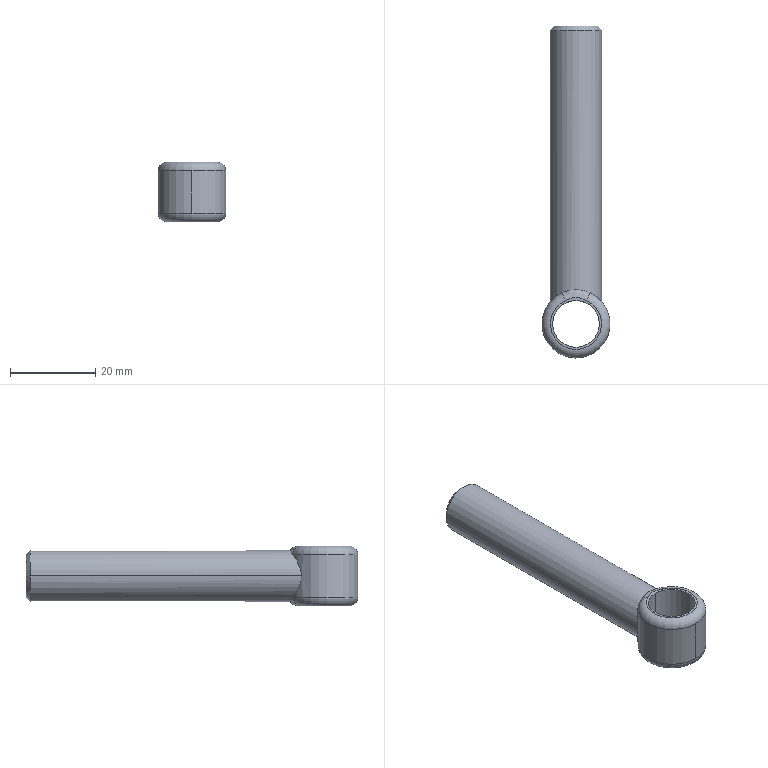Component | SolidWorks | LinkBolt-2 | 1 solid | 15 faces | box 16 x 78 x 14 mm | volume 8469 mm3 | cylinder 6 | plane 3 | cone 2 | torus 2 | spline 2 | commonest cylinder face diameters 11 x2 16 x2 12 x2
STEP:
#1=COLOUR_RGB('',0.7922,0.8196,0.9333);
#2=FILL_AREA_STYLE_COLOUR('',#1);
#3=FILL_AREA_STYLE('',(#2));
#4=SURFACE_STYLE_FILL_AREA(#3);
#5=SURFACE_SIDE_STYLE('',(#4));
#6=SURFACE_STYLE_USAGE(.BOTH.,#5);
#7=PRESENTATION_STYLE_ASSIGNMENT((#6));
#8=CARTESIAN_POINT('',(24.528,-9.567,-7.874));
#9=VERTEX_POINT('',#8);
#10=CARTESIAN_POINT('',(24.921,-9.567,-7.874));
#11=VERTEX_POINT('',#10);
#12=CARTESIAN_POINT('',(24.724,-9.567,-7.874));
#13=DIRECTION('',(-0.,1.,-0.));
#14=DIRECTION('',(-1.,0.,0.));
#15=AXIS2_PLACEMENT_3D('',#12,#13,#14);
#16=CIRCLE('',#15,0.1969);
#17=EDGE_CURVE('',#9,#11,#16,.T.);
#18=ORIENTED_EDGE('',*,*,#17,.F.);
#19=CARTESIAN_POINT('',(24.488,-9.606,-7.874));
#20=VERTEX_POINT('',#19);
#21=CARTESIAN_POINT('',(24.528,-9.567,-7.874));
#22=DIRECTION('',(-0.7071,-0.7071,0.));
#23=VECTOR('',#22,39.37);
#24=LINE('',#21,#23);
#25=EDGE_CURVE('',#9,#20,#24,.T.);
#26=ORIENTED_EDGE('',*,*,#25,.T.);
#27=CARTESIAN_POINT('',(24.961,-9.606,-7.874));
#28=VERTEX_POINT('',#27);
#29=CARTESIAN_POINT('',(24.724,-9.606,-7.874));
#30=DIRECTION('',(0.,-1.,0.));
#31=DIRECTION('',(-1.,0.,0.));
#32=AXIS2_PLACEMENT_3D('',#29,#30,#31);
#33=CIRCLE('',#32,0.2362);
#34=EDGE_CURVE('',#28,#20,#33,.T.);
#35=ORIENTED_EDGE('',*,*,#34,.F.);
#36=CARTESIAN_POINT('',(24.921,-9.567,-7.874));
#37=DIRECTION('',(0.7071,-0.7071,0.));
#38=VECTOR('',#37,39.37);
#39=LINE('',#36,#38);
#40=EDGE_CURVE('',#11,#28,#39,.T.);
#41=ORIENTED_EDGE('',*,*,#40,.F.);
#42=EDGE_LOOP('',(#18,#26,#35,#41));
#43=FACE_OUTER_BOUND('',#42,.T.);
#44=CARTESIAN_POINT('',(24.724,-9.567,-7.874));
#45=DIRECTION('',(0.,-1.,0.));
#46=DIRECTION('',(1.,0.,0.));
#47=AXIS2_PLACEMENT_3D('',#44,#45,#46);
#48=CONICAL_SURFACE('',#47,0.1969,0.7854);
#49=ADVANCED_FACE('',(#43),#48,.T.);
#50=CARTESIAN_POINT('',(24.724,-12.539,-8.15));
#51=VERTEX_POINT('',#50);
#52=CARTESIAN_POINT('',(24.724,-12.106,-8.15));
#53=VERTEX_POINT('',#52);
#54=CARTESIAN_POINT('',(24.724,-12.323,-8.15));
#55=DIRECTION('',(0.,0.,1.));
#56=DIRECTION('',(0.,1.,0.));
#57=AXIS2_PLACEMENT_3D('',#54,#55,#56);
#58=CIRCLE('',#57,0.2165);
#59=EDGE_CURVE('',#51,#53,#58,.T.);
#60=ORIENTED_EDGE('',*,*,#59,.F.);
#61=CARTESIAN_POINT('',(24.724,-12.539,-7.598));
#62=VERTEX_POINT('',#61);
#63=CARTESIAN_POINT('',(24.724,-12.539,-8.15));
#64=DIRECTION('',(0.,0.,1.));
#65=VECTOR('',#64,39.37);
#66=LINE('',#63,#65);
#67=EDGE_CURVE('',#51,#62,#66,.T.);
#68=ORIENTED_EDGE('',*,*,#67,.T.);
#69=CARTESIAN_POINT('',(24.724,-12.106,-7.598));
#70=VERTEX_POINT('',#69);
#71=CARTESIAN_POINT('',(24.724,-12.323,-7.598));
#72=DIRECTION('',(0.,0.,1.));
#73=DIRECTION('',(0.,1.,0.));
#74=AXIS2_PLACEMENT_3D('',#71,#72,#73);
#75=CIRCLE('',#74,0.2165);
#76=EDGE_CURVE('',#62,#70,#75,.T.);
#77=ORIENTED_EDGE('',*,*,#76,.T.);
#78=CARTESIAN_POINT('',(24.724,-12.106,-8.15));
#79=DIRECTION('',(0.,0.,1.));
#80=VECTOR('',#79,39.37);
#81=LINE('',#78,#80);
#82=EDGE_CURVE('',#53,#70,#81,.T.);
#83=ORIENTED_EDGE('',*,*,#82,.F.);
#84=EDGE_LOOP('',(#60,#68,#77,#83));
#85=FACE_OUTER_BOUND('',#84,.T.);
#86=CARTESIAN_POINT('',(24.724,-12.323,-8.15));
#87=DIRECTION('',(0.,0.,1.));
#88=DIRECTION('',(0.,1.,0.));
#89=AXIS2_PLACEMENT_3D('',#86,#87,#88);
#90=CYLINDRICAL_SURFACE('',#89,0.2165);
#91=ADVANCED_FACE('',(#85),#90,.F.);
#92=CARTESIAN_POINT('',(24.855,-12.036,-7.677));
#93=VERTEX_POINT('',#92);
#94=CARTESIAN_POINT('',(24.724,-12.638,-7.677));
#95=VERTEX_POINT('',#94);
#96=CARTESIAN_POINT('',(24.724,-12.323,-7.677));
#97=DIRECTION('',(0.,-0.,-1.));
#98=DIRECTION('',(0.,1.,0.));
#99=AXIS2_PLACEMENT_3D('',#96,#97,#98);
#100=CIRCLE('',#99,0.315);
#101=EDGE_CURVE('',#93,#95,#100,.T.);
#102=ORIENTED_EDGE('',*,*,#101,.T.);
#103=CARTESIAN_POINT('',(24.724,-12.638,-8.071));
#104=VERTEX_POINT('',#103);
#105=CARTESIAN_POINT('',(24.724,-12.638,-7.598));
#106=DIRECTION('',(0.,-0.,-1.));
#107=VECTOR('',#106,39.37);
#108=LINE('',#105,#107);
#109=EDGE_CURVE('',#95,#104,#108,.T.);
#110=ORIENTED_EDGE('',*,*,#109,.T.);
#111=CARTESIAN_POINT('',(24.855,-12.036,-8.071));
#112=VERTEX_POINT('',#111);
#113=CARTESIAN_POINT('',(24.724,-12.323,-8.071));
#114=DIRECTION('',(0.,0.,1.));
#115=DIRECTION('',(0.,1.,0.));
#116=AXIS2_PLACEMENT_3D('',#113,#114,#115);
#117=CIRCLE('',#116,0.315);
#118=EDGE_CURVE('',#104,#112,#117,.T.);
#119=ORIENTED_EDGE('',*,*,#118,.T.);
#120=CARTESIAN_POINT('',(24.961,-12.115,-7.874));
#121=VERTEX_POINT('',#120);
#122=CARTESIAN_POINT('',(24.855,-12.036,-8.071));
#123=CARTESIAN_POINT('',(24.863,-12.04,-8.066));
#124=CARTESIAN_POINT('',(24.871,-12.044,-8.06));
#125=CARTESIAN_POINT('',(24.885,-12.052,-8.047));
#126=CARTESIAN_POINT('',(24.892,-12.056,-8.041));
#127=CARTESIAN_POINT('',(24.911,-12.069,-8.02));
#128=CARTESIAN_POINT('',(24.922,-12.077,-8.005));
#129=CARTESIAN_POINT('',(24.936,-12.089,-7.98));
#130=CARTESIAN_POINT('',(24.94,-12.093,-7.971));
#131=CARTESIAN_POINT('',(24.947,-12.1,-7.953));
#132=CARTESIAN_POINT('',(24.95,-12.103,-7.944));
#133=CARTESIAN_POINT('',(24.955,-12.109,-7.925));
#134=CARTESIAN_POINT('',(24.957,-12.111,-7.915));
#135=CARTESIAN_POINT('',(24.96,-12.114,-7.895));
#136=CARTESIAN_POINT('',(24.961,-12.115,-7.884));
#137=CARTESIAN_POINT('',(24.961,-12.115,-7.874));
#138=B_SPLINE_CURVE_WITH_KNOTS('',3,(#122,#123,#124,#125,#126,#127,#128,#129,#130,#131,#132,#133,#134,#135,#136,#137),.UNSPECIFIED.,.F.,.F.,(4,2,2,2,2,2,2,4),(0.03295,0.03373,0.0345,0.03606,0.03683,0.03761,0.03838,0.03916),.UNSPECIFIED.);
#139=EDGE_CURVE('',#112,#121,#138,.T.);
#140=ORIENTED_EDGE('',*,*,#139,.T.);
#141=CARTESIAN_POINT('',(24.961,-12.115,-7.874));
#142=CARTESIAN_POINT('',(24.961,-12.115,-7.853));
#143=CARTESIAN_POINT('',(24.958,-12.111,-7.833));
#144=CARTESIAN_POINT('',(24.95,-12.103,-7.804));
#145=CARTESIAN_POINT('',(24.947,-12.1,-7.795));
#146=CARTESIAN_POINT('',(24.94,-12.093,-7.777));
#147=CARTESIAN_POINT('',(24.936,-12.089,-7.768));
#148=CARTESIAN_POINT('',(24.927,-12.081,-7.751));
#149=CARTESIAN_POINT('',(24.921,-12.077,-7.743));
#150=CARTESIAN_POINT('',(24.91,-12.069,-7.728));
#151=CARTESIAN_POINT('',(24.905,-12.064,-7.721));
#152=CARTESIAN_POINT('',(24.892,-12.056,-7.707));
#153=CARTESIAN_POINT('',(24.885,-12.052,-7.701));
#154=CARTESIAN_POINT('',(24.871,-12.044,-7.688));
#155=CARTESIAN_POINT('',(24.863,-12.04,-7.682));
#156=CARTESIAN_POINT('',(24.855,-12.036,-7.677));
#157=B_SPLINE_CURVE_WITH_KNOTS('',3,(#141,#142,#143,#144,#145,#146,#147,#148,#149,#150,#151,#152,#153,#154,#155,#156),.UNSPECIFIED.,.F.,.F.,(4,2,2,2,2,2,2,4),(0.,0.001558,0.002336,0.003115,0.003894,0.004673,0.005452,0.00623),.UNSPECIFIED.);
#158=EDGE_CURVE('',#121,#93,#157,.T.);
#159=ORIENTED_EDGE('',*,*,#158,.T.);
#160=EDGE_LOOP('',(#102,#110,#119,#140,#159));
#161=FACE_OUTER_BOUND('',#160,.T.);
#162=CARTESIAN_POINT('',(24.724,-12.323,-7.598));
#163=DIRECTION('',(0.,-0.,-1.));
#164=DIRECTION('',(0.,-1.,0.));
#165=AXIS2_PLACEMENT_3D('',#162,#163,#164);
#166=CYLINDRICAL_SURFACE('',#165,0.315);
#167=ADVANCED_FACE('',(#161),#166,.T.);
#168=ORIENTED_EDGE('',*,*,#34,.T.);
#169=CARTESIAN_POINT('',(24.488,-12.115,-7.874));
#170=VERTEX_POINT('',#169);
#171=CARTESIAN_POINT('',(24.488,-9.567,-7.874));
#172=DIRECTION('',(0.,-1.,0.));
#173=VECTOR('',#172,39.37);
#174=LINE('',#171,#173);
#175=EDGE_CURVE('',#20,#170,#174,.T.);
#176=ORIENTED_EDGE('',*,*,#175,.T.);
#177=CARTESIAN_POINT('',(24.594,-12.036,-7.677));
#178=VERTEX_POINT('',#177);
#179=CARTESIAN_POINT('',(24.594,-12.036,-7.677));
#180=CARTESIAN_POINT('',(24.586,-12.04,-7.682));
#181=CARTESIAN_POINT('',(24.578,-12.044,-7.688));
#182=CARTESIAN_POINT('',(24.564,-12.052,-7.701));
#183=CARTESIAN_POINT('',(24.557,-12.056,-7.707));
#184=CARTESIAN_POINT('',(24.538,-12.069,-7.728));
#185=CARTESIAN_POINT('',(24.527,-12.077,-7.743));
#186=CARTESIAN_POINT('',(24.513,-12.089,-7.768));
#187=CARTESIAN_POINT('',(24.509,-12.093,-7.777));
#188=CARTESIAN_POINT('',(24.502,-12.1,-7.795));
#189=CARTESIAN_POINT('',(24.499,-12.103,-7.804));
#190=CARTESIAN_POINT('',(24.494,-12.109,-7.823));
#191=CARTESIAN_POINT('',(24.492,-12.111,-7.833));
#192=CARTESIAN_POINT('',(24.489,-12.114,-7.853));
#193=CARTESIAN_POINT('',(24.488,-12.115,-7.864));
#194=CARTESIAN_POINT('',(24.488,-12.115,-7.874));
#195=B_SPLINE_CURVE_WITH_KNOTS('',3,(#179,#180,#181,#182,#183,#184,#185,#186,#187,#188,#189,#190,#191,#192,#193,#194),.UNSPECIFIED.,.F.,.F.,(4,2,2,2,2,2,2,4),(0.01338,0.01416,0.01494,0.01649,0.01727,0.01804,0.01882,0.0196),.UNSPECIFIED.);
#196=EDGE_CURVE('',#178,#170,#195,.T.);
#197=ORIENTED_EDGE('',*,*,#196,.F.);
#198=CARTESIAN_POINT('',(24.855,-12.036,-7.677));
#199=CARTESIAN_POINT('',(24.846,-12.032,-7.671));
#200=CARTESIAN_POINT('',(24.836,-12.028,-7.666));
#201=CARTESIAN_POINT('',(24.816,-12.021,-7.656));
#202=CARTESIAN_POINT('',(24.805,-12.018,-7.652));
#203=CARTESIAN_POINT('',(24.783,-12.013,-7.645));
#204=CARTESIAN_POINT('',(24.772,-12.011,-7.642));
#205=CARTESIAN_POINT('',(24.748,-12.009,-7.639));
#206=CARTESIAN_POINT('',(24.736,-12.008,-7.638));
#207=CARTESIAN_POINT('',(24.713,-12.008,-7.638));
#208=CARTESIAN_POINT('',(24.701,-12.009,-7.639));
#209=CARTESIAN_POINT('',(24.678,-12.011,-7.642));
#210=CARTESIAN_POINT('',(24.666,-12.013,-7.645));
#211=CARTESIAN_POINT('',(24.644,-12.018,-7.652));
#212=CARTESIAN_POINT('',(24.633,-12.021,-7.656));
#213=CARTESIAN_POINT('',(24.613,-12.028,-7.665));
#214=CARTESIAN_POINT('',(24.603,-12.032,-7.671));
#215=CARTESIAN_POINT('',(24.594,-12.036,-7.677));
#216=B_SPLINE_CURVE_WITH_KNOTS('',3,(#198,#199,#200,#201,#202,#203,#204,#205,#206,#207,#208,#209,#210,#211,#212,#213,#214,#215),.UNSPECIFIED.,.F.,.F.,(4,2,2,2,2,2,2,2,4),(0.00623,0.007124,0.008018,0.008912,0.009806,0.0107,0.01159,0.01249,0.01338),.UNSPECIFIED.);
#217=EDGE_CURVE('',#93,#178,#216,.T.);
#218=ORIENTED_EDGE('',*,*,#217,.F.);
#219=ORIENTED_EDGE('',*,*,#158,.F.);
#220=CARTESIAN_POINT('',(24.961,-9.567,-7.874));
#221=DIRECTION('',(0.,-1.,0.));
#222=VECTOR('',#221,39.37);
#223=LINE('',#220,#222);
#224=EDGE_CURVE('',#28,#121,#223,.T.);
#225=ORIENTED_EDGE('',*,*,#224,.F.);
#226=EDGE_LOOP('',(#168,#176,#197,#218,#219,#225));
#227=FACE_OUTER_BOUND('',#226,.T.);
#228=CARTESIAN_POINT('',(24.724,-9.567,-7.874));
#229=DIRECTION('',(0.,-1.,0.));
#230=DIRECTION('',(1.,0.,0.));
#231=AXIS2_PLACEMENT_3D('',#228,#229,#230);
#232=CYLINDRICAL_SURFACE('',#231,0.2362);
#233=ADVANCED_FACE('',(#227),#232,.T.);
#234=ORIENTED_EDGE('',*,*,#175,.F.);
#235=CARTESIAN_POINT('',(24.724,-9.606,-7.874));
#236=DIRECTION('',(0.,-1.,0.));
#237=DIRECTION('',(-1.,0.,0.));
#238=AXIS2_PLACEMENT_3D('',#235,#236,#237);
#239=CIRCLE('',#238,0.2362);
#240=EDGE_CURVE('',#20,#28,#239,.T.);
#241=ORIENTED_EDGE('',*,*,#240,.T.);
#242=ORIENTED_EDGE('',*,*,#224,.T.);
#243=ORIENTED_EDGE('',*,*,#139,.F.);
#244=CARTESIAN_POINT('',(24.594,-12.036,-8.071));
#245=VERTEX_POINT('',#244);
#246=CARTESIAN_POINT('',(24.594,-12.036,-8.071));
#247=CARTESIAN_POINT('',(24.603,-12.032,-8.077));
#248=CARTESIAN_POINT('',(24.613,-12.028,-8.082));
#249=CARTESIAN_POINT('',(24.633,-12.021,-8.092));
#250=CARTESIAN_POINT('',(24.644,-12.018,-8.096));
#251=CARTESIAN_POINT('',(24.666,-12.013,-8.103));
#252=CARTESIAN_POINT('',(24.677,-12.011,-8.106));
#253=CARTESIAN_POINT('',(24.7,-12.009,-8.109));
#254=CARTESIAN_POINT('',(24.712,-12.008,-8.11));
#255=CARTESIAN_POINT('',(24.736,-12.008,-8.11));
#256=CARTESIAN_POINT('',(24.748,-12.009,-8.109));
#257=CARTESIAN_POINT('',(24.771,-12.011,-8.106));
#258=CARTESIAN_POINT('',(24.783,-12.013,-8.103));
#259=CARTESIAN_POINT('',(24.805,-12.018,-8.096));
#260=CARTESIAN_POINT('',(24.815,-12.021,-8.092));
#261=CARTESIAN_POINT('',(24.836,-12.028,-8.083));
#262=CARTESIAN_POINT('',(24.846,-12.032,-8.077));
#263=CARTESIAN_POINT('',(24.855,-12.036,-8.071));
#264=B_SPLINE_CURVE_WITH_KNOTS('',3,(#246,#247,#248,#249,#250,#251,#252,#253,#254,#255,#256,#257,#258,#259,#260,#261,#262,#263),.UNSPECIFIED.,.F.,.F.,(4,2,2,2,2,2,2,2,4),(0.02581,0.02671,0.0276,0.02849,0.02938,0.03028,0.03117,0.03206,0.03295),.UNSPECIFIED.);
#265=EDGE_CURVE('',#245,#112,#264,.T.);
#266=ORIENTED_EDGE('',*,*,#265,.F.);
#267=CARTESIAN_POINT('',(24.488,-12.115,-7.874));
#268=CARTESIAN_POINT('',(24.488,-12.115,-7.884));
#269=CARTESIAN_POINT('',(24.489,-12.114,-7.895));
#270=CARTESIAN_POINT('',(24.492,-12.111,-7.915));
#271=CARTESIAN_POINT('',(24.494,-12.109,-7.925));
#272=CARTESIAN_POINT('',(24.501,-12.1,-7.954));
#273=CARTESIAN_POINT('',(24.508,-12.093,-7.972));
#274=CARTESIAN_POINT('',(24.522,-12.081,-7.997));
#275=CARTESIAN_POINT('',(24.527,-12.077,-8.005));
#276=CARTESIAN_POINT('',(24.538,-12.069,-8.02));
#277=CARTESIAN_POINT('',(24.544,-12.064,-8.027));
#278=CARTESIAN_POINT('',(24.563,-12.052,-8.048));
#279=CARTESIAN_POINT('',(24.578,-12.043,-8.06));
#280=CARTESIAN_POINT('',(24.594,-12.036,-8.071));
#281=B_SPLINE_CURVE_WITH_KNOTS('',3,(#267,#268,#269,#270,#271,#272,#273,#274,#275,#276,#277,#278,#279,#280),.UNSPECIFIED.,.F.,.F.,(4,2,2,2,2,2,4),(0.0196,0.02037,0.02115,0.02271,0.02348,0.02426,0.02581),.UNSPECIFIED.);
#282=EDGE_CURVE('',#170,#245,#281,.T.);
#283=ORIENTED_EDGE('',*,*,#282,.F.);
#284=EDGE_LOOP('',(#234,#241,#242,#243,#266,#283));
#285=FACE_OUTER_BOUND('',#284,.T.);
#286=CARTESIAN_POINT('',(24.724,-9.567,-7.874));
#287=DIRECTION('',(0.,-1.,0.));
#288=DIRECTION('',(1.,0.,0.));
#289=AXIS2_PLACEMENT_3D('',#286,#287,#288);
#290=CYLINDRICAL_SURFACE('',#289,0.2362);
#291=ADVANCED_FACE('',(#285),#290,.T.);
#292=CARTESIAN_POINT('',(24.724,-9.567,-7.874));
#293=DIRECTION('',(-0.,1.,-0.));
#294=DIRECTION('',(-1.,0.,0.));
#295=AXIS2_PLACEMENT_3D('',#292,#293,#294);
#296=CIRCLE('',#295,0.1969);
#297=EDGE_CURVE('',#11,#9,#296,.T.);
#298=ORIENTED_EDGE('',*,*,#297,.T.);
#299=ORIENTED_EDGE('',*,*,#17,.T.);
#300=EDGE_LOOP('',(#298,#299));
#301=FACE_OUTER_BOUND('',#300,.T.);
#302=CARTESIAN_POINT('',(24.724,-9.567,-7.874));
#303=DIRECTION('',(-0.,1.,-0.));
#304=DIRECTION('',(-1.,-0.,0.));
#305=AXIS2_PLACEMENT_3D('',#302,#303,#304);
#306=PLANE('',#305);
#307=ADVANCED_FACE('',(#301),#306,.T.);
#308=ORIENTED_EDGE('',*,*,#109,.F.);
#309=CARTESIAN_POINT('',(24.724,-12.323,-7.677));
#310=DIRECTION('',(0.,-0.,-1.));
#311=DIRECTION('',(0.,1.,0.));
#312=AXIS2_PLACEMENT_3D('',#309,#310,#311);
#313=CIRCLE('',#312,0.315);
#314=EDGE_CURVE('',#95,#178,#313,.T.);
#315=ORIENTED_EDGE('',*,*,#314,.T.);
#316=ORIENTED_EDGE('',*,*,#196,.T.);
#317=ORIENTED_EDGE('',*,*,#282,.T.);
#318=CARTESIAN_POINT('',(24.724,-12.323,-8.071));
#319=DIRECTION('',(0.,0.,1.));
#320=DIRECTION('',(0.,1.,0.));
#321=AXIS2_PLACEMENT_3D('',#318,#319,#320);
#322=CIRCLE('',#321,0.315);
#323=EDGE_CURVE('',#245,#104,#322,.T.);
#324=ORIENTED_EDGE('',*,*,#323,.T.);
#325=EDGE_LOOP('',(#308,#315,#316,#317,#324));
#326=FACE_OUTER_BOUND('',#325,.T.);
#327=CARTESIAN_POINT('',(24.724,-12.323,-7.598));
#328=DIRECTION('',(0.,-0.,-1.));
#329=DIRECTION('',(0.,-1.,0.));
#330=AXIS2_PLACEMENT_3D('',#327,#328,#329);
#331=CYLINDRICAL_SURFACE('',#330,0.315);
#332=ADVANCED_FACE('',(#326),#331,.T.);
#333=CARTESIAN_POINT('',(24.626,-12.108,-7.598));
#334=VERTEX_POINT('',#333);
#335=CARTESIAN_POINT('',(24.822,-12.108,-7.598));
#336=VERTEX_POINT('',#335);
#337=CARTESIAN_POINT('',(24.724,-12.323,-7.598));
#338=DIRECTION('',(0.,0.,1.));
#339=DIRECTION('',(0.,1.,0.));
#340=AXIS2_PLACEMENT_3D('',#337,#338,#339);
#341=CIRCLE('',#340,0.2362);
#342=EDGE_CURVE('',#334,#336,#341,.T.);
#343=ORIENTED_EDGE('',*,*,#342,.T.);
#344=CARTESIAN_POINT('',(24.822,-12.108,-7.598));
#345=CARTESIAN_POINT('',(24.807,-12.101,-7.598));
#346=CARTESIAN_POINT('',(24.791,-12.093,-7.598));
#347=CARTESIAN_POINT('',(24.759,-12.08,-7.598));
#348=CARTESIAN_POINT('',(24.742,-12.076,-7.598));
#349=CARTESIAN_POINT('',(24.716,-12.076,-7.598));
#350=CARTESIAN_POINT('',(24.707,-12.077,-7.598));
#351=CARTESIAN_POINT('',(24.69,-12.081,-7.598));
#352=CARTESIAN_POINT('',(24.682,-12.084,-7.598));
#353=CARTESIAN_POINT('',(24.658,-12.093,-7.598));
#354=CARTESIAN_POINT('',(24.642,-12.101,-7.598));
#355=CARTESIAN_POINT('',(24.626,-12.108,-7.598));
#356=B_SPLINE_CURVE_WITH_KNOTS('',3,(#344,#345,#346,#347,#348,#349,#350,#351,#352,#353,#354,#355),.UNSPECIFIED.,.F.,.F.,(4,2,2,2,2,4),(0.,0.001321,0.002643,0.003303,0.003964,0.005286),.UNSPECIFIED.);
#357=EDGE_CURVE('',#336,#334,#356,.T.);
#358=ORIENTED_EDGE('',*,*,#357,.T.);
#359=EDGE_LOOP('',(#343,#358));
#360=FACE_OUTER_BOUND('',#359,.T.);
#361=CARTESIAN_POINT('',(24.724,-12.323,-7.598));
#362=DIRECTION('',(0.,0.,1.));
#363=DIRECTION('',(0.,1.,0.));
#364=AXIS2_PLACEMENT_3D('',#361,#362,#363);
#365=CIRCLE('',#364,0.2165);
#366=EDGE_CURVE('',#70,#62,#365,.T.);
#367=ORIENTED_EDGE('',*,*,#366,.F.);
#368=ORIENTED_EDGE('',*,*,#76,.F.);
#369=EDGE_LOOP('',(#367,#368));
#370=FACE_BOUND('',#369,.T.);
#371=CARTESIAN_POINT('',(24.724,-12.323,-7.598));
#372=DIRECTION('',(-0.,0.,1.));
#373=DIRECTION('',(-0.,1.,-0.));
#374=AXIS2_PLACEMENT_3D('',#371,#372,#373);
#375=PLANE('',#374);
#376=ADVANCED_FACE('',(#360,#370),#375,.T.);
#377=CARTESIAN_POINT('',(24.626,-12.108,-8.15));
#378=VERTEX_POINT('',#377);
#379=CARTESIAN_POINT('',(24.822,-12.108,-8.15));
#380=VERTEX_POINT('',#379);
#381=CARTESIAN_POINT('',(24.626,-12.108,-8.15));
#382=CARTESIAN_POINT('',(24.642,-12.101,-8.15));
#383=CARTESIAN_POINT('',(24.658,-12.093,-8.15));
#384=CARTESIAN_POINT('',(24.69,-12.08,-8.15));
#385=CARTESIAN_POINT('',(24.707,-12.076,-8.15));
#386=CARTESIAN_POINT('',(24.733,-12.076,-8.15));
#387=CARTESIAN_POINT('',(24.742,-12.077,-8.15));
#388=CARTESIAN_POINT('',(24.758,-12.081,-8.15));
#389=CARTESIAN_POINT('',(24.767,-12.084,-8.15));
#390=CARTESIAN_POINT('',(24.791,-12.093,-8.15));
#391=CARTESIAN_POINT('',(24.807,-12.101,-8.15));
#392=CARTESIAN_POINT('',(24.822,-12.108,-8.15));
#393=B_SPLINE_CURVE_WITH_KNOTS('',3,(#381,#382,#383,#384,#385,#386,#387,#388,#389,#390,#391,#392),.UNSPECIFIED.,.F.,.F.,(4,2,2,2,2,4),(0.,0.001321,0.002643,0.003303,0.003964,0.005286),.UNSPECIFIED.);
#394=EDGE_CURVE('',#378,#380,#393,.T.);
#395=ORIENTED_EDGE('',*,*,#394,.T.);
#396=CARTESIAN_POINT('',(24.724,-12.323,-8.15));
#397=DIRECTION('',(0.,-0.,-1.));
#398=DIRECTION('',(0.,1.,0.));
#399=AXIS2_PLACEMENT_3D('',#396,#397,#398);
#400=CIRCLE('',#399,0.2362);
#401=EDGE_CURVE('',#380,#378,#400,.T.);
#402=ORIENTED_EDGE('',*,*,#401,.T.);
#403=EDGE_LOOP('',(#395,#402));
#404=FACE_OUTER_BOUND('',#403,.T.);
#405=CARTESIAN_POINT('',(24.724,-12.323,-8.15));
#406=DIRECTION('',(0.,0.,1.));
#407=DIRECTION('',(0.,1.,0.));
#408=AXIS2_PLACEMENT_3D('',#405,#406,#407);
#409=CIRCLE('',#408,0.2165);
#410=EDGE_CURVE('',#53,#51,#409,.T.);
#411=ORIENTED_EDGE('',*,*,#410,.T.);
#412=ORIENTED_EDGE('',*,*,#59,.T.);
#413=EDGE_LOOP('',(#411,#412));
#414=FACE_BOUND('',#413,.T.);
#415=CARTESIAN_POINT('',(24.724,-12.323,-8.15));
#416=DIRECTION('',(-0.,0.,1.));
#417=DIRECTION('',(-0.,1.,-0.));
#418=AXIS2_PLACEMENT_3D('',#415,#416,#417);
#419=PLANE('',#418);
#420=ADVANCED_FACE('',(#404,#414),#419,.F.);
#421=ORIENTED_EDGE('',*,*,#67,.F.);
#422=ORIENTED_EDGE('',*,*,#410,.F.);
#423=ORIENTED_EDGE('',*,*,#82,.T.);
#424=ORIENTED_EDGE('',*,*,#366,.T.);
#425=EDGE_LOOP('',(#421,#422,#423,#424));
#426=FACE_OUTER_BOUND('',#425,.T.);
#427=CARTESIAN_POINT('',(24.724,-12.323,-8.15));
#428=DIRECTION('',(0.,0.,1.));
#429=DIRECTION('',(0.,1.,0.));
#430=AXIS2_PLACEMENT_3D('',#427,#428,#429);
#431=CYLINDRICAL_SURFACE('',#430,0.2165);
#432=ADVANCED_FACE('',(#426),#431,.F.);
#433=CARTESIAN_POINT('',(24.626,-12.108,-8.071));
#434=DIRECTION('',(0.91,0.4146,-0.));
#435=DIRECTION('',(-0.4146,0.91,0.));
#436=AXIS2_PLACEMENT_3D('',#433,#434,#435);
#437=CIRCLE('',#436,0.07874);
#438=EDGE_CURVE('',#378,#245,#437,.T.);
#439=ORIENTED_EDGE('',*,*,#438,.F.);
#440=ORIENTED_EDGE('',*,*,#401,.F.);
#441=CARTESIAN_POINT('',(24.822,-12.108,-8.071));
#442=DIRECTION('',(-0.91,0.4146,-0.));
#443=DIRECTION('',(-0.4146,-0.91,0.));
#444=AXIS2_PLACEMENT_3D('',#441,#442,#443);
#445=CIRCLE('',#444,0.07874);
#446=EDGE_CURVE('',#112,#380,#445,.T.);
#447=ORIENTED_EDGE('',*,*,#446,.F.);
#448=ORIENTED_EDGE('',*,*,#118,.F.);
#449=ORIENTED_EDGE('',*,*,#323,.F.);
#450=EDGE_LOOP('',(#439,#440,#447,#448,#449));
#451=FACE_OUTER_BOUND('',#450,.T.);
#452=CARTESIAN_POINT('',(24.724,-12.323,-8.071));
#453=DIRECTION('',(0.,0.,1.));
#454=DIRECTION('',(0.,1.,-0.));
#455=AXIS2_PLACEMENT_3D('',#452,#453,#454);
#456=TOROIDAL_SURFACE('',#455,0.2362,0.07874);
#457=ADVANCED_FACE('',(#451),#456,.T.);
#458=ORIENTED_EDGE('',*,*,#446,.T.);
#459=ORIENTED_EDGE('',*,*,#394,.F.);
#460=ORIENTED_EDGE('',*,*,#438,.T.);
#461=ORIENTED_EDGE('',*,*,#265,.T.);
#462=EDGE_LOOP('',(#458,#459,#460,#461));
#463=FACE_OUTER_BOUND('',#462,.T.);
#464=CARTESIAN_POINT('',(24.822,-12.108,-8.15));
#465=CARTESIAN_POINT('',(24.855,-12.036,-8.15));
#466=CARTESIAN_POINT('',(24.855,-12.036,-8.071));
#467=CARTESIAN_POINT('',(24.807,-12.101,-8.15));
#468=CARTESIAN_POINT('',(24.838,-12.038,-8.15));
#469=CARTESIAN_POINT('',(24.841,-12.03,-8.08));
#470=CARTESIAN_POINT('',(24.791,-12.093,-8.15));
#471=CARTESIAN_POINT('',(24.818,-12.037,-8.15));
#472=CARTESIAN_POINT('',(24.823,-12.023,-8.09));
#473=CARTESIAN_POINT('',(24.767,-12.084,-8.15));
#474=CARTESIAN_POINT('',(24.784,-12.034,-8.15));
#475=CARTESIAN_POINT('',(24.79,-12.015,-8.101));
#476=CARTESIAN_POINT('',(24.758,-12.081,-8.15));
#477=CARTESIAN_POINT('',(24.772,-12.033,-8.15));
#478=CARTESIAN_POINT('',(24.778,-12.012,-8.104));
#479=CARTESIAN_POINT('',(24.742,-12.077,-8.15));
#480=CARTESIAN_POINT('',(24.749,-12.031,-8.15));
#481=CARTESIAN_POINT('',(24.752,-12.009,-8.109));
#482=CARTESIAN_POINT('',(24.733,-12.076,-8.15));
#483=CARTESIAN_POINT('',(24.737,-12.031,-8.15));
#484=CARTESIAN_POINT('',(24.739,-12.008,-8.11));
#485=CARTESIAN_POINT('',(24.716,-12.076,-8.15));
#486=CARTESIAN_POINT('',(24.712,-12.031,-8.15));
#487=CARTESIAN_POINT('',(24.71,-12.008,-8.11));
#488=CARTESIAN_POINT('',(24.707,-12.077,-8.15));
#489=CARTESIAN_POINT('',(24.7,-12.031,-8.15));
#490=CARTESIAN_POINT('',(24.696,-12.009,-8.109));
#491=CARTESIAN_POINT('',(24.69,-12.081,-8.15));
#492=CARTESIAN_POINT('',(24.676,-12.033,-8.15));
#493=CARTESIAN_POINT('',(24.67,-12.012,-8.104));
#494=CARTESIAN_POINT('',(24.682,-12.084,-8.15));
#495=CARTESIAN_POINT('',(24.665,-12.034,-8.15));
#496=CARTESIAN_POINT('',(24.658,-12.015,-8.101));
#497=CARTESIAN_POINT('',(24.658,-12.093,-8.15));
#498=CARTESIAN_POINT('',(24.631,-12.037,-8.15));
#499=CARTESIAN_POINT('',(24.625,-12.023,-8.09));
#500=CARTESIAN_POINT('',(24.642,-12.101,-8.15));
#501=CARTESIAN_POINT('',(24.611,-12.038,-8.15));
#502=CARTESIAN_POINT('',(24.608,-12.03,-8.08));
#503=CARTESIAN_POINT('',(24.626,-12.108,-8.15));
#504=CARTESIAN_POINT('',(24.594,-12.036,-8.15));
#505=CARTESIAN_POINT('',(24.594,-12.036,-8.071));
#506=(BOUNDED_SURFACE()B_SPLINE_SURFACE(3,2,((#464,#465,#466),(#467,#468,#469),(#470,#471,#472),(#473,#474,#475),(#476,#477,#478),(#479,#480,#481),(#482,#483,#484),(#485,#486,#487),(#488,#489,#490),(#491,#492,#493),(#494,#495,#496),(#497,#498,#499),(#500,#501,#502),(#503,#504,#505)),.UNSPECIFIED.,.F.,.F.,.T.)B_SPLINE_SURFACE_WITH_KNOTS((4,2,2,2,2,2,4),(3,3),(0.003735,0.005052,0.00571,0.006369,0.007027,0.007685,0.009002),(0.,1.),.UNSPECIFIED.)GEOMETRIC_REPRESENTATION_ITEM()RATIONAL_B_SPLINE_SURFACE(((1.,0.7071,1.),(1.,0.7491,1.),(1.,0.7879,1.),(1.,0.8321,1.),(1.,0.8443,1.),(1.,0.8613,1.),(1.,0.866,1.),(1.,0.866,1.),(1.,0.8613,1.),(1.,0.8443,1.),(1.,0.8321,1.),(1.,0.7879,1.),(1.,0.7491,1.),(1.,0.7071,1.)))REPRESENTATION_ITEM('')SURFACE());
#507=ADVANCED_FACE('',(#463),#506,.T.);
#508=CARTESIAN_POINT('',(24.626,-12.108,-7.677));
#509=DIRECTION('',(0.91,0.4146,-0.));
#510=DIRECTION('',(-0.4146,0.91,0.));
#511=AXIS2_PLACEMENT_3D('',#508,#509,#510);
#512=CIRCLE('',#511,0.07874);
#513=EDGE_CURVE('',#178,#334,#512,.T.);
#514=ORIENTED_EDGE('',*,*,#513,.F.);
#515=ORIENTED_EDGE('',*,*,#314,.F.);
#516=ORIENTED_EDGE('',*,*,#101,.F.);
#517=CARTESIAN_POINT('',(24.822,-12.108,-7.677));
#518=DIRECTION('',(-0.91,0.4146,-0.));
#519=DIRECTION('',(-0.4146,-0.91,0.));
#520=AXIS2_PLACEMENT_3D('',#517,#518,#519);
#521=CIRCLE('',#520,0.07874);
#522=EDGE_CURVE('',#336,#93,#521,.T.);
#523=ORIENTED_EDGE('',*,*,#522,.F.);
#524=ORIENTED_EDGE('',*,*,#342,.F.);
#525=EDGE_LOOP('',(#514,#515,#516,#523,#524));
#526=FACE_OUTER_BOUND('',#525,.T.);
#527=CARTESIAN_POINT('',(24.724,-12.323,-7.677));
#528=DIRECTION('',(0.,0.,1.));
#529=DIRECTION('',(0.,1.,-0.));
#530=AXIS2_PLACEMENT_3D('',#527,#528,#529);
#531=TOROIDAL_SURFACE('',#530,0.2362,0.07874);
#532=ADVANCED_FACE('',(#526),#531,.T.);
#533=ORIENTED_EDGE('',*,*,#522,.T.);
#534=ORIENTED_EDGE('',*,*,#217,.T.);
#535=ORIENTED_EDGE('',*,*,#513,.T.);
#536=ORIENTED_EDGE('',*,*,#357,.F.);
#537=EDGE_LOOP('',(#533,#534,#535,#536));
#538=FACE_OUTER_BOUND('',#537,.T.);
#539=CARTESIAN_POINT('',(24.626,-12.108,-7.598));
#540=CARTESIAN_POINT('',(24.594,-12.036,-7.598));
#541=CARTESIAN_POINT('',(24.594,-12.036,-7.677));
#542=CARTESIAN_POINT('',(24.642,-12.101,-7.598));
#543=CARTESIAN_POINT('',(24.611,-12.038,-7.598));
#544=CARTESIAN_POINT('',(24.608,-12.03,-7.668));
#545=CARTESIAN_POINT('',(24.658,-12.093,-7.598));
#546=CARTESIAN_POINT('',(24.631,-12.037,-7.598));
#547=CARTESIAN_POINT('',(24.625,-12.023,-7.658));
#548=CARTESIAN_POINT('',(24.682,-12.084,-7.598));
#549=CARTESIAN_POINT('',(24.665,-12.034,-7.598));
#550=CARTESIAN_POINT('',(24.658,-12.015,-7.647));
#551=CARTESIAN_POINT('',(24.69,-12.081,-7.598));
#552=CARTESIAN_POINT('',(24.676,-12.033,-7.598));
#553=CARTESIAN_POINT('',(24.671,-12.012,-7.644));
#554=CARTESIAN_POINT('',(24.707,-12.077,-7.598));
#555=CARTESIAN_POINT('',(24.7,-12.031,-7.598));
#556=CARTESIAN_POINT('',(24.696,-12.009,-7.639));
#557=CARTESIAN_POINT('',(24.716,-12.076,-7.598));
#558=CARTESIAN_POINT('',(24.712,-12.031,-7.598));
#559=CARTESIAN_POINT('',(24.71,-12.008,-7.638));
#560=CARTESIAN_POINT('',(24.733,-12.076,-7.598));
#561=CARTESIAN_POINT('',(24.737,-12.031,-7.598));
#562=CARTESIAN_POINT('',(24.739,-12.008,-7.638));
#563=CARTESIAN_POINT('',(24.742,-12.077,-7.598));
#564=CARTESIAN_POINT('',(24.749,-12.031,-7.598));
#565=CARTESIAN_POINT('',(24.752,-12.009,-7.639));
#566=CARTESIAN_POINT('',(24.758,-12.081,-7.598));
#567=CARTESIAN_POINT('',(24.772,-12.033,-7.598));
#568=CARTESIAN_POINT('',(24.778,-12.012,-7.644));
#569=CARTESIAN_POINT('',(24.767,-12.084,-7.598));
#570=CARTESIAN_POINT('',(24.784,-12.034,-7.598));
#571=CARTESIAN_POINT('',(24.79,-12.015,-7.647));
#572=CARTESIAN_POINT('',(24.791,-12.093,-7.598));
#573=CARTESIAN_POINT('',(24.818,-12.037,-7.598));
#574=CARTESIAN_POINT('',(24.823,-12.023,-7.658));
#575=CARTESIAN_POINT('',(24.807,-12.101,-7.598));
#576=CARTESIAN_POINT('',(24.838,-12.038,-7.598));
#577=CARTESIAN_POINT('',(24.841,-12.03,-7.668));
#578=CARTESIAN_POINT('',(24.822,-12.108,-7.598));
#579=CARTESIAN_POINT('',(24.855,-12.036,-7.598));
#580=CARTESIAN_POINT('',(24.855,-12.036,-7.677));
#581=(BOUNDED_SURFACE()B_SPLINE_SURFACE(3,2,((#539,#540,#541),(#542,#543,#544),(#545,#546,#547),(#548,#549,#550),(#551,#552,#553),(#554,#555,#556),(#557,#558,#559),(#560,#561,#562),(#563,#564,#565),(#566,#567,#568),(#569,#570,#571),(#572,#573,#574),(#575,#576,#577),(#578,#579,#580)),.UNSPECIFIED.,.F.,.F.,.F.)B_SPLINE_SURFACE_WITH_KNOTS((4,2,2,2,2,2,4),(3,3),(0.003735,0.005052,0.00571,0.006369,0.007027,0.007685,0.009002),(0.,1.),.UNSPECIFIED.)GEOMETRIC_REPRESENTATION_ITEM()RATIONAL_B_SPLINE_SURFACE(((1.,0.7071,1.),(1.,0.7491,1.),(1.,0.7879,1.),(1.,0.8321,1.),(1.,0.8443,1.),(1.,0.8613,1.),(1.,0.866,1.),(1.,0.866,1.),(1.,0.8613,1.),(1.,0.8443,1.),(1.,0.8321,1.),(1.,0.7879,1.),(1.,0.7491,1.),(1.,0.7071,1.)))REPRESENTATION_ITEM('')SURFACE());
#582=ADVANCED_FACE('',(#538),#581,.T.);
#583=ORIENTED_EDGE('',*,*,#25,.F.);
#584=ORIENTED_EDGE('',*,*,#297,.F.);
#585=ORIENTED_EDGE('',*,*,#40,.T.);
#586=ORIENTED_EDGE('',*,*,#240,.F.);
#587=EDGE_LOOP('',(#583,#584,#585,#586));
#588=FACE_OUTER_BOUND('',#587,.T.);
#589=CARTESIAN_POINT('',(24.724,-9.567,-7.874));
#590=DIRECTION('',(0.,-1.,0.));
#591=DIRECTION('',(1.,0.,0.));
#592=AXIS2_PLACEMENT_3D('',#589,#590,#591);
#593=CONICAL_SURFACE('',#592,0.1969,0.7854);
#594=ADVANCED_FACE('',(#588),#593,.T.);
#595=CLOSED_SHELL('',(#49,#91,#167,#233,#291,#307,#332,#376,#420,#432,#457,#507,#532,#582,#594));
#596=MANIFOLD_SOLID_BREP('',#595);
#597=STYLED_ITEM('',(#7),#596);
#598=PRESENTATION_LAYER_ASSIGNMENT('','',(#597));
#599=CARTESIAN_POINT('',(0.,0.,0.));
#600=DIRECTION('',(0.,0.,1.));
#601=DIRECTION('',(1.,0.,0.));
#602=AXIS2_PLACEMENT_3D('',#599,#600,#601);
#603=(LENGTH_UNIT()NAMED_UNIT(*)SI_UNIT($,.METRE.));
#604=LENGTH_MEASURE_WITH_UNIT(LENGTH_MEASURE(0.0254),#603);
#605=DIMENSIONAL_EXPONENTS(1.,0.,0.,0.,0.,0.,0.);
#606=(CONVERSION_BASED_UNIT('',#604)LENGTH_UNIT()NAMED_UNIT(#605));
#607=UNCERTAINTY_MEASURE_WITH_UNIT(LENGTH_MEASURE(0.00001),#606,'','');
#608=(NAMED_UNIT(*)PLANE_ANGLE_UNIT()SI_UNIT($,.RADIAN.));
#609=(NAMED_UNIT(*)SI_UNIT($,.STERADIAN.)SOLID_ANGLE_UNIT());
#610=(GEOMETRIC_REPRESENTATION_CONTEXT(3)GLOBAL_UNCERTAINTY_ASSIGNED_CONTEXT((#607))GLOBAL_UNIT_ASSIGNED_CONTEXT((#606,#608,#609))REPRESENTATION_CONTEXT('',''));
#611=ADVANCED_BREP_SHAPE_REPRESENTATION('',(#596,#602),#610);
#612=(LENGTH_UNIT()NAMED_UNIT(*)SI_UNIT($,.METRE.));
#613=LENGTH_MEASURE_WITH_UNIT(LENGTH_MEASURE(0.0254),#612);
#614=DIMENSIONAL_EXPONENTS(1.,0.,0.,0.,0.,0.,0.);
#615=(CONVERSION_BASED_UNIT('',#613)LENGTH_UNIT()NAMED_UNIT(#614));
#616=UNCERTAINTY_MEASURE_WITH_UNIT(LENGTH_MEASURE(0.00001),#615,'','');
#617=(NAMED_UNIT(*)PLANE_ANGLE_UNIT()SI_UNIT($,.RADIAN.));
#618=(NAMED_UNIT(*)SI_UNIT($,.STERADIAN.)SOLID_ANGLE_UNIT());
#619=(GEOMETRIC_REPRESENTATION_CONTEXT(3)GLOBAL_UNCERTAINTY_ASSIGNED_CONTEXT((#616))GLOBAL_UNIT_ASSIGNED_CONTEXT((#615,#617,#618))REPRESENTATION_CONTEXT('',''));
#620=MECHANICAL_DESIGN_GEOMETRIC_PRESENTATION_REPRESENTATION('',(#597),#619);